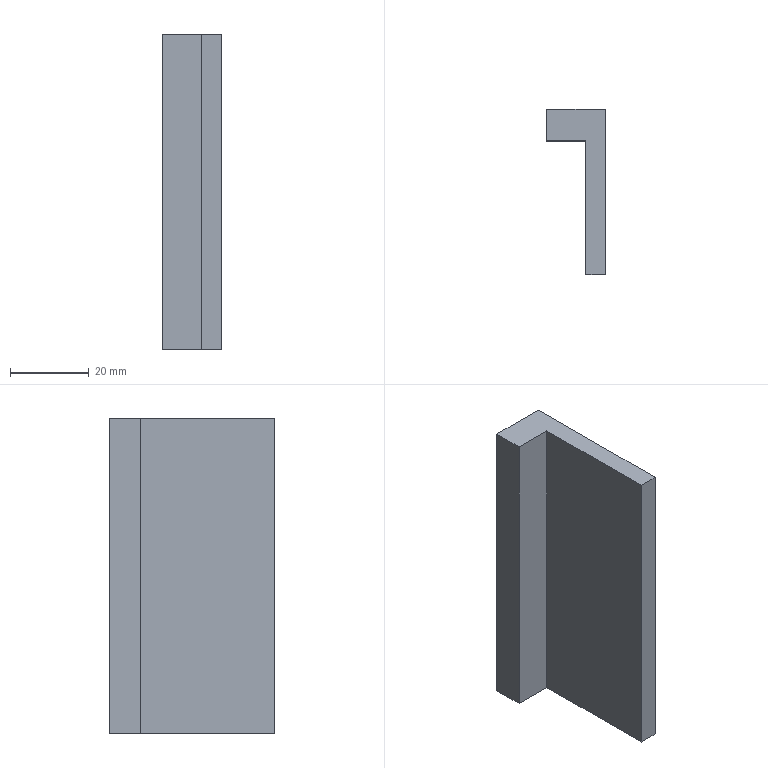Component | SolidWorks | Inline-H010-H01160308-005K-1 | 1 solid | 8 faces | box 15 x 42 x 80 mm | volume 23200 mm3 | plane 8
build123d program:
from build123d import *

# Parameters (mm, degrees)
BOSS_EXTRUDE1_DEPTH = 40


with BuildPart() as part:
    # Sketch1 → Boss-Extrude1 (new, symmetric)
    with BuildSketch(Plane.XY):
        Polygon((0, 0), (0, 42), (15, 42), (15, 34), (5, 34), (5, 0), align=None)
    extrude(amount=BOSS_EXTRUDE1_DEPTH, both=True)


solid = part.part

# Placed as in the assembly
solid = solid.moved(Location((68.768, -4.032, 132.262), (-180, 0, 180)))
STEP:
#1=COLOUR_RGB('',0.7922,0.8196,0.9333);
#2=FILL_AREA_STYLE_COLOUR('',#1);
#3=FILL_AREA_STYLE('',(#2));
#4=SURFACE_STYLE_FILL_AREA(#3);
#5=SURFACE_SIDE_STYLE('',(#4));
#6=SURFACE_STYLE_USAGE(.BOTH.,#5);
#7=PRESENTATION_STYLE_ASSIGNMENT((#6));
#8=CARTESIAN_POINT('',(2.707,-0.1588,6.782));
#9=VERTEX_POINT('',#8);
#10=CARTESIAN_POINT('',(2.511,-0.1588,6.782));
#11=VERTEX_POINT('',#10);
#12=CARTESIAN_POINT('',(2.511,-0.1588,6.782));
#13=DIRECTION('',(-1.,0.,0.));
#14=VECTOR('',#13,39.37);
#15=LINE('',#12,#14);
#16=EDGE_CURVE('',#9,#11,#15,.T.);
#17=ORIENTED_EDGE('',*,*,#16,.T.);
#18=CARTESIAN_POINT('',(2.511,-0.1588,3.632));
#19=VERTEX_POINT('',#18);
#20=CARTESIAN_POINT('',(2.511,-0.1588,3.632));
#21=DIRECTION('',(0.,-0.,1.));
#22=VECTOR('',#21,39.37);
#23=LINE('',#20,#22);
#24=EDGE_CURVE('',#19,#11,#23,.T.);
#25=ORIENTED_EDGE('',*,*,#24,.F.);
#26=CARTESIAN_POINT('',(2.707,-0.1588,3.632));
#27=VERTEX_POINT('',#26);
#28=CARTESIAN_POINT('',(2.511,-0.1588,3.632));
#29=DIRECTION('',(-1.,0.,0.));
#30=VECTOR('',#29,39.37);
#31=LINE('',#28,#30);
#32=EDGE_CURVE('',#27,#19,#31,.T.);
#33=ORIENTED_EDGE('',*,*,#32,.F.);
#34=CARTESIAN_POINT('',(2.707,-0.1588,3.632));
#35=DIRECTION('',(0.,-0.,1.));
#36=VECTOR('',#35,39.37);
#37=LINE('',#34,#36);
#38=EDGE_CURVE('',#27,#9,#37,.T.);
#39=ORIENTED_EDGE('',*,*,#38,.T.);
#40=EDGE_LOOP('',(#17,#25,#33,#39));
#41=FACE_OUTER_BOUND('',#40,.T.);
#42=CARTESIAN_POINT('',(2.511,-0.1588,3.632));
#43=DIRECTION('',(0.,1.,0.));
#44=DIRECTION('',(1.,-0.,-0.));
#45=AXIS2_PLACEMENT_3D('',#42,#43,#44);
#46=PLANE('',#45);
#47=ADVANCED_FACE('',(#41),#46,.F.);
#48=CARTESIAN_POINT('',(2.511,1.18,6.782));
#49=VERTEX_POINT('',#48);
#50=CARTESIAN_POINT('',(2.511,1.18,6.782));
#51=DIRECTION('',(0.,1.,0.));
#52=VECTOR('',#51,39.37);
#53=LINE('',#50,#52);
#54=EDGE_CURVE('',#11,#49,#53,.T.);
#55=ORIENTED_EDGE('',*,*,#54,.T.);
#56=CARTESIAN_POINT('',(2.511,1.18,3.632));
#57=VERTEX_POINT('',#56);
#58=CARTESIAN_POINT('',(2.511,1.18,3.632));
#59=DIRECTION('',(0.,-0.,1.));
#60=VECTOR('',#59,39.37);
#61=LINE('',#58,#60);
#62=EDGE_CURVE('',#57,#49,#61,.T.);
#63=ORIENTED_EDGE('',*,*,#62,.F.);
#64=CARTESIAN_POINT('',(2.511,1.18,3.632));
#65=DIRECTION('',(0.,1.,0.));
#66=VECTOR('',#65,39.37);
#67=LINE('',#64,#66);
#68=EDGE_CURVE('',#19,#57,#67,.T.);
#69=ORIENTED_EDGE('',*,*,#68,.F.);
#70=ORIENTED_EDGE('',*,*,#24,.T.);
#71=EDGE_LOOP('',(#55,#63,#69,#70));
#72=FACE_OUTER_BOUND('',#71,.T.);
#73=CARTESIAN_POINT('',(2.511,1.18,3.632));
#74=DIRECTION('',(1.,-0.,-0.));
#75=DIRECTION('',(-0.,-1.,-0.));
#76=AXIS2_PLACEMENT_3D('',#73,#74,#75);
#77=PLANE('',#76);
#78=ADVANCED_FACE('',(#72),#77,.F.);
#79=CARTESIAN_POINT('',(2.117,1.18,6.782));
#80=VERTEX_POINT('',#79);
#81=CARTESIAN_POINT('',(2.117,1.18,6.782));
#82=DIRECTION('',(-1.,0.,0.));
#83=VECTOR('',#82,39.37);
#84=LINE('',#81,#83);
#85=EDGE_CURVE('',#49,#80,#84,.T.);
#86=ORIENTED_EDGE('',*,*,#85,.T.);
#87=CARTESIAN_POINT('',(2.117,1.18,3.632));
#88=VERTEX_POINT('',#87);
#89=CARTESIAN_POINT('',(2.117,1.18,3.632));
#90=DIRECTION('',(0.,-0.,1.));
#91=VECTOR('',#90,39.37);
#92=LINE('',#89,#91);
#93=EDGE_CURVE('',#88,#80,#92,.T.);
#94=ORIENTED_EDGE('',*,*,#93,.F.);
#95=CARTESIAN_POINT('',(2.117,1.18,3.632));
#96=DIRECTION('',(-1.,0.,0.));
#97=VECTOR('',#96,39.37);
#98=LINE('',#95,#97);
#99=EDGE_CURVE('',#57,#88,#98,.T.);
#100=ORIENTED_EDGE('',*,*,#99,.F.);
#101=ORIENTED_EDGE('',*,*,#62,.T.);
#102=EDGE_LOOP('',(#86,#94,#100,#101));
#103=FACE_OUTER_BOUND('',#102,.T.);
#104=CARTESIAN_POINT('',(2.117,1.18,3.632));
#105=DIRECTION('',(0.,1.,0.));
#106=DIRECTION('',(-0.,0.,-1.));
#107=AXIS2_PLACEMENT_3D('',#104,#105,#106);
#108=PLANE('',#107);
#109=ADVANCED_FACE('',(#103),#108,.F.);
#110=CARTESIAN_POINT('',(2.117,1.495,6.782));
#111=VERTEX_POINT('',#110);
#112=CARTESIAN_POINT('',(2.117,1.495,6.782));
#113=DIRECTION('',(0.,1.,0.));
#114=VECTOR('',#113,39.37);
#115=LINE('',#112,#114);
#116=EDGE_CURVE('',#80,#111,#115,.T.);
#117=ORIENTED_EDGE('',*,*,#116,.T.);
#118=CARTESIAN_POINT('',(2.117,1.495,3.632));
#119=VERTEX_POINT('',#118);
#120=CARTESIAN_POINT('',(2.117,1.495,3.632));
#121=DIRECTION('',(0.,-0.,1.));
#122=VECTOR('',#121,39.37);
#123=LINE('',#120,#122);
#124=EDGE_CURVE('',#119,#111,#123,.T.);
#125=ORIENTED_EDGE('',*,*,#124,.F.);
#126=CARTESIAN_POINT('',(2.117,1.495,3.632));
#127=DIRECTION('',(0.,1.,0.));
#128=VECTOR('',#127,39.37);
#129=LINE('',#126,#128);
#130=EDGE_CURVE('',#88,#119,#129,.T.);
#131=ORIENTED_EDGE('',*,*,#130,.F.);
#132=ORIENTED_EDGE('',*,*,#93,.T.);
#133=EDGE_LOOP('',(#117,#125,#131,#132));
#134=FACE_OUTER_BOUND('',#133,.T.);
#135=CARTESIAN_POINT('',(2.117,1.495,3.632));
#136=DIRECTION('',(1.,-0.,-0.));
#137=DIRECTION('',(-0.,0.,-1.));
#138=AXIS2_PLACEMENT_3D('',#135,#136,#137);
#139=PLANE('',#138);
#140=ADVANCED_FACE('',(#134),#139,.F.);
#141=CARTESIAN_POINT('',(2.707,1.495,6.782));
#142=VERTEX_POINT('',#141);
#143=CARTESIAN_POINT('',(2.707,1.495,6.782));
#144=DIRECTION('',(1.,-0.,-0.));
#145=VECTOR('',#144,39.37);
#146=LINE('',#143,#145);
#147=EDGE_CURVE('',#111,#142,#146,.T.);
#148=ORIENTED_EDGE('',*,*,#147,.T.);
#149=CARTESIAN_POINT('',(2.707,1.495,3.632));
#150=VERTEX_POINT('',#149);
#151=CARTESIAN_POINT('',(2.707,1.495,3.632));
#152=DIRECTION('',(0.,-0.,1.));
#153=VECTOR('',#152,39.37);
#154=LINE('',#151,#153);
#155=EDGE_CURVE('',#150,#142,#154,.T.);
#156=ORIENTED_EDGE('',*,*,#155,.F.);
#157=CARTESIAN_POINT('',(2.707,1.495,3.632));
#158=DIRECTION('',(1.,-0.,-0.));
#159=VECTOR('',#158,39.37);
#160=LINE('',#157,#159);
#161=EDGE_CURVE('',#119,#150,#160,.T.);
#162=ORIENTED_EDGE('',*,*,#161,.F.);
#163=ORIENTED_EDGE('',*,*,#124,.T.);
#164=EDGE_LOOP('',(#148,#156,#162,#163));
#165=FACE_OUTER_BOUND('',#164,.T.);
#166=CARTESIAN_POINT('',(2.707,1.495,3.632));
#167=DIRECTION('',(-0.,-1.,-0.));
#168=DIRECTION('',(0.,-0.,1.));
#169=AXIS2_PLACEMENT_3D('',#166,#167,#168);
#170=PLANE('',#169);
#171=ADVANCED_FACE('',(#165),#170,.F.);
#172=CARTESIAN_POINT('',(2.707,-0.1588,6.782));
#173=DIRECTION('',(-0.,-1.,-0.));
#174=VECTOR('',#173,39.37);
#175=LINE('',#172,#174);
#176=EDGE_CURVE('',#142,#9,#175,.T.);
#177=ORIENTED_EDGE('',*,*,#176,.T.);
#178=ORIENTED_EDGE('',*,*,#38,.F.);
#179=CARTESIAN_POINT('',(2.707,-0.1588,3.632));
#180=DIRECTION('',(-0.,-1.,-0.));
#181=VECTOR('',#180,39.37);
#182=LINE('',#179,#181);
#183=EDGE_CURVE('',#150,#27,#182,.T.);
#184=ORIENTED_EDGE('',*,*,#183,.F.);
#185=ORIENTED_EDGE('',*,*,#155,.T.);
#186=EDGE_LOOP('',(#177,#178,#184,#185));
#187=FACE_OUTER_BOUND('',#186,.T.);
#188=CARTESIAN_POINT('',(2.707,-0.1588,3.632));
#189=DIRECTION('',(-1.,0.,0.));
#190=DIRECTION('',(0.,-0.,1.));
#191=AXIS2_PLACEMENT_3D('',#188,#189,#190);
#192=PLANE('',#191);
#193=ADVANCED_FACE('',(#187),#192,.F.);
#194=ORIENTED_EDGE('',*,*,#32,.T.);
#195=ORIENTED_EDGE('',*,*,#68,.T.);
#196=ORIENTED_EDGE('',*,*,#99,.T.);
#197=ORIENTED_EDGE('',*,*,#130,.T.);
#198=ORIENTED_EDGE('',*,*,#161,.T.);
#199=ORIENTED_EDGE('',*,*,#183,.T.);
#200=EDGE_LOOP('',(#194,#195,#196,#197,#198,#199));
#201=FACE_OUTER_BOUND('',#200,.T.);
#202=CARTESIAN_POINT('',(2.707,-0.1588,3.632));
#203=DIRECTION('',(0.,-0.,1.));
#204=DIRECTION('',(1.,-0.,-0.));
#205=AXIS2_PLACEMENT_3D('',#202,#203,#204);
#206=PLANE('',#205);
#207=ADVANCED_FACE('',(#201),#206,.F.);
#208=ORIENTED_EDGE('',*,*,#16,.F.);
#209=ORIENTED_EDGE('',*,*,#176,.F.);
#210=ORIENTED_EDGE('',*,*,#147,.F.);
#211=ORIENTED_EDGE('',*,*,#116,.F.);
#212=ORIENTED_EDGE('',*,*,#85,.F.);
#213=ORIENTED_EDGE('',*,*,#54,.F.);
#214=EDGE_LOOP('',(#208,#209,#210,#211,#212,#213));
#215=FACE_OUTER_BOUND('',#214,.T.);
#216=CARTESIAN_POINT('',(2.707,-0.1588,6.782));
#217=DIRECTION('',(0.,-0.,1.));
#218=DIRECTION('',(1.,-0.,-0.));
#219=AXIS2_PLACEMENT_3D('',#216,#217,#218);
#220=PLANE('',#219);
#221=ADVANCED_FACE('',(#215),#220,.T.);
#222=CLOSED_SHELL('',(#47,#78,#109,#140,#171,#193,#207,#221));
#223=MANIFOLD_SOLID_BREP('',#222);
#224=STYLED_ITEM('',(#7),#223);
#225=(LENGTH_UNIT()NAMED_UNIT(*)SI_UNIT($,.METRE.));
#226=LENGTH_MEASURE_WITH_UNIT(LENGTH_MEASURE(0.0254),#225);
#227=DIMENSIONAL_EXPONENTS(1.,0.,0.,0.,0.,0.,0.);
#228=(CONVERSION_BASED_UNIT('',#226)LENGTH_UNIT()NAMED_UNIT(#227));
#229=UNCERTAINTY_MEASURE_WITH_UNIT(LENGTH_MEASURE(0.00001),#228,'','');
#230=(NAMED_UNIT(*)PLANE_ANGLE_UNIT()SI_UNIT($,.RADIAN.));
#231=(NAMED_UNIT(*)SI_UNIT($,.STERADIAN.)SOLID_ANGLE_UNIT());
#232=(GEOMETRIC_REPRESENTATION_CONTEXT(3)GLOBAL_UNCERTAINTY_ASSIGNED_CONTEXT((#229))GLOBAL_UNIT_ASSIGNED_CONTEXT((#228,#230,#231))REPRESENTATION_CONTEXT('',''));
#233=MECHANICAL_DESIGN_GEOMETRIC_PRESENTATION_REPRESENTATION('',(#224),#232);
#234=CARTESIAN_POINT('',(0.,0.,0.));
#235=DIRECTION('',(0.,0.,1.));
#236=DIRECTION('',(1.,0.,0.));
#237=AXIS2_PLACEMENT_3D('',#234,#235,#236);
#238=(LENGTH_UNIT()NAMED_UNIT(*)SI_UNIT($,.METRE.));
#239=LENGTH_MEASURE_WITH_UNIT(LENGTH_MEASURE(0.0254),#238);
#240=DIMENSIONAL_EXPONENTS(1.,0.,0.,0.,0.,0.,0.);
#241=(CONVERSION_BASED_UNIT('',#239)LENGTH_UNIT()NAMED_UNIT(#240));
#242=UNCERTAINTY_MEASURE_WITH_UNIT(LENGTH_MEASURE(0.00001),#241,'','');
#243=(NAMED_UNIT(*)PLANE_ANGLE_UNIT()SI_UNIT($,.RADIAN.));
#244=(NAMED_UNIT(*)SI_UNIT($,.STERADIAN.)SOLID_ANGLE_UNIT());
#245=(GEOMETRIC_REPRESENTATION_CONTEXT(3)GLOBAL_UNCERTAINTY_ASSIGNED_CONTEXT((#242))GLOBAL_UNIT_ASSIGNED_CONTEXT((#241,#243,#244))REPRESENTATION_CONTEXT('',''));
#246=ADVANCED_BREP_SHAPE_REPRESENTATION('',(#223,#237),#245);
#247=PRESENTATION_LAYER_ASSIGNMENT('','',(#224));